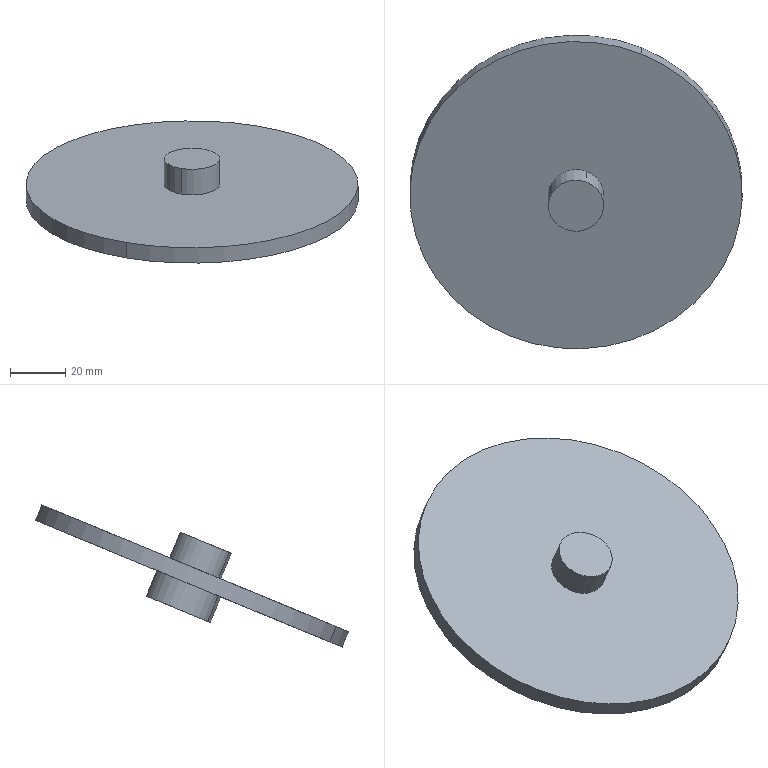Component | SolidWorks | EccentricWheel-2 | 1 solid | 10 faces | box 120 x 113.2 x 51.37 mm | volume 75909 mm3 | cylinder 6 | plane 4 | commonest cylinder face diameters 20 x2 25 x2 120 x2
build123d program:
from build123d import *

# Parameters (mm, degrees)
SKETCH1_R           = 60
BOSS_EXTRUDE1_DEPTH = 6
SKETCH2_R           = 12.5
BOSS_EXTRUDE2_DEPTH = 10
SKETCH3_R           = 10
BOSS_EXTRUDE3_DEPTH = 10


with BuildPart() as part:
    # Sketch1 → Boss-Extrude1 (new body)
    with BuildSketch(Plane.XY):
        Circle(SKETCH1_R)
    extrude(amount=BOSS_EXTRUDE1_DEPTH)

    # Sketch2 → Boss-Extrude2 (add)
    with BuildSketch(Plane(origin=(0, 0, 0), x_dir=(-1, 0, 0), z_dir=(0, 0, -1))):
        Circle(SKETCH2_R)
    extrude(amount=BOSS_EXTRUDE2_DEPTH)

    # Sketch3 → Boss-Extrude3 (add)
    with BuildSketch(Plane.XY.offset(6)):
        Circle(SKETCH3_R)
    extrude(amount=BOSS_EXTRUDE3_DEPTH)


solid = part.part

# Placed as in the assembly
solid = solid.moved(Location((-36.329, 4.513, 6.427), (22.448, 0, 0)))
STEP:
#1=COLOUR_RGB('',0.7922,0.8196,0.9333);
#2=FILL_AREA_STYLE_COLOUR('',#1);
#3=FILL_AREA_STYLE('',(#2));
#4=SURFACE_STYLE_FILL_AREA(#3);
#5=SURFACE_SIDE_STYLE('',(#4));
#6=SURFACE_STYLE_USAGE(.BOTH.,#5);
#7=PRESENTATION_STYLE_ASSIGNMENT((#6));
#8=CARTESIAN_POINT('',(-1.586,-0.3971,0.6971));
#9=VERTEX_POINT('',#8);
#10=CARTESIAN_POINT('',(-1.275,0.2714,0.9733));
#11=VERTEX_POINT('',#10);
#12=CARTESIAN_POINT('',(-1.43,-0.06285,0.8352));
#13=DIRECTION('',(0.,-0.3818,0.9242));
#14=DIRECTION('',(-0.3951,-0.849,-0.3508));
#15=AXIS2_PLACEMENT_3D('',#12,#13,#14);
#16=CIRCLE('',#15,0.3937);
#17=EDGE_CURVE('',#9,#11,#16,.T.);
#18=ORIENTED_EDGE('',*,*,#17,.F.);
#19=CARTESIAN_POINT('',(-1.586,-0.2468,0.3332));
#20=VERTEX_POINT('',#19);
#21=CARTESIAN_POINT('',(-1.586,-0.3971,0.6971));
#22=DIRECTION('',(-0.,0.3818,-0.9242));
#23=VECTOR('',#22,39.37);
#24=LINE('',#21,#23);
#25=EDGE_CURVE('',#9,#20,#24,.T.);
#26=ORIENTED_EDGE('',*,*,#25,.T.);
#27=CARTESIAN_POINT('',(-1.275,0.4218,0.6095));
#28=VERTEX_POINT('',#27);
#29=CARTESIAN_POINT('',(-1.43,0.08749,0.4714));
#30=DIRECTION('',(0.,-0.3818,0.9242));
#31=DIRECTION('',(-0.3951,-0.849,-0.3508));
#32=AXIS2_PLACEMENT_3D('',#29,#30,#31);
#33=CIRCLE('',#32,0.3937);
#34=EDGE_CURVE('',#20,#28,#33,.T.);
#35=ORIENTED_EDGE('',*,*,#34,.T.);
#36=CARTESIAN_POINT('',(-1.275,0.2714,0.9733));
#37=DIRECTION('',(-0.,0.3818,-0.9242));
#38=VECTOR('',#37,39.37);
#39=LINE('',#36,#38);
#40=EDGE_CURVE('',#11,#28,#39,.T.);
#41=ORIENTED_EDGE('',*,*,#40,.F.);
#42=EDGE_LOOP('',(#18,#26,#35,#41));
#43=FACE_OUTER_BOUND('',#42,.T.);
#44=CARTESIAN_POINT('',(-1.43,-0.06285,0.8352));
#45=DIRECTION('',(-0.,0.3818,-0.9242));
#46=DIRECTION('',(0.3951,0.849,0.3508));
#47=AXIS2_PLACEMENT_3D('',#44,#45,#46);
#48=CYLINDRICAL_SURFACE('',#47,0.3937);
#49=ADVANCED_FACE('',(#43),#48,.T.);
#50=CARTESIAN_POINT('',(-1.236,0.7459,0.0618));
#51=VERTEX_POINT('',#50);
#52=CARTESIAN_POINT('',(-1.625,-0.08981,-0.2835));
#53=VERTEX_POINT('',#52);
#54=CARTESIAN_POINT('',(-1.43,0.328,-0.1108));
#55=DIRECTION('',(-0.,0.3818,-0.9242));
#56=DIRECTION('',(0.3951,0.849,0.3508));
#57=AXIS2_PLACEMENT_3D('',#54,#55,#56);
#58=CIRCLE('',#57,0.4921);
#59=EDGE_CURVE('',#51,#53,#58,.T.);
#60=ORIENTED_EDGE('',*,*,#59,.F.);
#61=CARTESIAN_POINT('',(-1.236,0.5955,0.4257));
#62=VERTEX_POINT('',#61);
#63=CARTESIAN_POINT('',(-1.236,0.7459,0.0618));
#64=DIRECTION('',(0.,-0.3818,0.9242));
#65=VECTOR('',#64,39.37);
#66=LINE('',#63,#65);
#67=EDGE_CURVE('',#51,#62,#66,.T.);
#68=ORIENTED_EDGE('',*,*,#67,.T.);
#69=CARTESIAN_POINT('',(-1.625,-0.2401,0.0804));
#70=VERTEX_POINT('',#69);
#71=CARTESIAN_POINT('',(-1.43,0.1777,0.253));
#72=DIRECTION('',(-0.,0.3818,-0.9242));
#73=DIRECTION('',(0.3951,0.849,0.3508));
#74=AXIS2_PLACEMENT_3D('',#71,#72,#73);
#75=CIRCLE('',#74,0.4921);
#76=EDGE_CURVE('',#62,#70,#75,.T.);
#77=ORIENTED_EDGE('',*,*,#76,.T.);
#78=CARTESIAN_POINT('',(-1.625,-0.08981,-0.2835));
#79=DIRECTION('',(0.,-0.3818,0.9242));
#80=VECTOR('',#79,39.37);
#81=LINE('',#78,#80);
#82=EDGE_CURVE('',#53,#70,#81,.T.);
#83=ORIENTED_EDGE('',*,*,#82,.F.);
#84=EDGE_LOOP('',(#60,#68,#77,#83));
#85=FACE_OUTER_BOUND('',#84,.T.);
#86=CARTESIAN_POINT('',(-1.43,0.328,-0.1108));
#87=DIRECTION('',(0.,-0.3818,0.9242));
#88=DIRECTION('',(-0.3951,-0.849,-0.3508));
#89=AXIS2_PLACEMENT_3D('',#86,#87,#88);
#90=CYLINDRICAL_SURFACE('',#89,0.4921);
#91=ADVANCED_FACE('',(#85),#90,.T.);
#92=CARTESIAN_POINT('',(-2.364,-1.918,-0.3573));
#93=VERTEX_POINT('',#92);
#94=CARTESIAN_POINT('',(-0.497,2.093,1.3));
#95=VERTEX_POINT('',#94);
#96=CARTESIAN_POINT('',(-1.43,0.08749,0.4714));
#97=DIRECTION('',(0.,-0.3818,0.9242));
#98=DIRECTION('',(-0.3951,-0.849,-0.3508));
#99=AXIS2_PLACEMENT_3D('',#96,#97,#98);
#100=CIRCLE('',#99,2.362);
#101=EDGE_CURVE('',#93,#95,#100,.T.);
#102=ORIENTED_EDGE('',*,*,#101,.F.);
#103=CARTESIAN_POINT('',(-2.364,-1.828,-0.5756));
#104=VERTEX_POINT('',#103);
#105=CARTESIAN_POINT('',(-2.364,-1.918,-0.3573));
#106=DIRECTION('',(-0.,0.3818,-0.9242));
#107=VECTOR('',#106,39.37);
#108=LINE('',#105,#107);
#109=EDGE_CURVE('',#93,#104,#108,.T.);
#110=ORIENTED_EDGE('',*,*,#109,.T.);
#111=CARTESIAN_POINT('',(-0.497,2.183,1.082));
#112=VERTEX_POINT('',#111);
#113=CARTESIAN_POINT('',(-1.43,0.1777,0.253));
#114=DIRECTION('',(0.,-0.3818,0.9242));
#115=DIRECTION('',(-0.3951,-0.849,-0.3508));
#116=AXIS2_PLACEMENT_3D('',#113,#114,#115);
#117=CIRCLE('',#116,2.362);
#118=EDGE_CURVE('',#104,#112,#117,.T.);
#119=ORIENTED_EDGE('',*,*,#118,.T.);
#120=CARTESIAN_POINT('',(-0.497,2.093,1.3));
#121=DIRECTION('',(-0.,0.3818,-0.9242));
#122=VECTOR('',#121,39.37);
#123=LINE('',#120,#122);
#124=EDGE_CURVE('',#95,#112,#123,.T.);
#125=ORIENTED_EDGE('',*,*,#124,.F.);
#126=EDGE_LOOP('',(#102,#110,#119,#125));
#127=FACE_OUTER_BOUND('',#126,.T.);
#128=CARTESIAN_POINT('',(-1.43,0.08749,0.4714));
#129=DIRECTION('',(-0.,0.3818,-0.9242));
#130=DIRECTION('',(0.3951,0.849,0.3508));
#131=AXIS2_PLACEMENT_3D('',#128,#129,#130);
#132=CYLINDRICAL_SURFACE('',#131,2.362);
#133=ADVANCED_FACE('',(#127),#132,.T.);
#134=ORIENTED_EDGE('',*,*,#109,.F.);
#135=CARTESIAN_POINT('',(-1.43,0.08749,0.4714));
#136=DIRECTION('',(0.,-0.3818,0.9242));
#137=DIRECTION('',(-0.3951,-0.849,-0.3508));
#138=AXIS2_PLACEMENT_3D('',#135,#136,#137);
#139=CIRCLE('',#138,2.362);
#140=EDGE_CURVE('',#95,#93,#139,.T.);
#141=ORIENTED_EDGE('',*,*,#140,.F.);
#142=ORIENTED_EDGE('',*,*,#124,.T.);
#143=CARTESIAN_POINT('',(-1.43,0.1777,0.253));
#144=DIRECTION('',(0.,-0.3818,0.9242));
#145=DIRECTION('',(-0.3951,-0.849,-0.3508));
#146=AXIS2_PLACEMENT_3D('',#143,#144,#145);
#147=CIRCLE('',#146,2.362);
#148=EDGE_CURVE('',#112,#104,#147,.T.);
#149=ORIENTED_EDGE('',*,*,#148,.T.);
#150=EDGE_LOOP('',(#134,#141,#142,#149));
#151=FACE_OUTER_BOUND('',#150,.T.);
#152=CARTESIAN_POINT('',(-1.43,0.08749,0.4714));
#153=DIRECTION('',(-0.,0.3818,-0.9242));
#154=DIRECTION('',(0.3951,0.849,0.3508));
#155=AXIS2_PLACEMENT_3D('',#152,#153,#154);
#156=CYLINDRICAL_SURFACE('',#155,2.362);
#157=ADVANCED_FACE('',(#151),#156,.T.);
#158=CARTESIAN_POINT('',(-1.43,0.08749,0.4714));
#159=DIRECTION('',(0.,-0.3818,0.9242));
#160=DIRECTION('',(-0.3951,-0.849,-0.3508));
#161=AXIS2_PLACEMENT_3D('',#158,#159,#160);
#162=CIRCLE('',#161,0.3937);
#163=EDGE_CURVE('',#28,#20,#162,.T.);
#164=ORIENTED_EDGE('',*,*,#163,.F.);
#165=ORIENTED_EDGE('',*,*,#34,.F.);
#166=EDGE_LOOP('',(#164,#165));
#167=FACE_BOUND('',#166,.T.);
#168=ORIENTED_EDGE('',*,*,#140,.T.);
#169=ORIENTED_EDGE('',*,*,#101,.T.);
#170=EDGE_LOOP('',(#168,#169));
#171=FACE_OUTER_BOUND('',#170,.T.);
#172=CARTESIAN_POINT('',(-1.43,0.08749,0.4714));
#173=DIRECTION('',(0.,-0.3818,0.9242));
#174=DIRECTION('',(-0.3951,-0.849,-0.3508));
#175=AXIS2_PLACEMENT_3D('',#172,#173,#174);
#176=PLANE('',#175);
#177=ADVANCED_FACE('',(#167,#171),#176,.T.);
#178=CARTESIAN_POINT('',(-1.43,0.1777,0.253));
#179=DIRECTION('',(-0.,0.3818,-0.9242));
#180=DIRECTION('',(0.3951,0.849,0.3508));
#181=AXIS2_PLACEMENT_3D('',#178,#179,#180);
#182=CIRCLE('',#181,0.4921);
#183=EDGE_CURVE('',#70,#62,#182,.T.);
#184=ORIENTED_EDGE('',*,*,#183,.F.);
#185=ORIENTED_EDGE('',*,*,#76,.F.);
#186=EDGE_LOOP('',(#184,#185));
#187=FACE_BOUND('',#186,.T.);
#188=ORIENTED_EDGE('',*,*,#148,.F.);
#189=ORIENTED_EDGE('',*,*,#118,.F.);
#190=EDGE_LOOP('',(#188,#189));
#191=FACE_OUTER_BOUND('',#190,.T.);
#192=CARTESIAN_POINT('',(-1.43,0.1777,0.253));
#193=DIRECTION('',(0.,-0.3818,0.9242));
#194=DIRECTION('',(-0.3951,-0.849,-0.3508));
#195=AXIS2_PLACEMENT_3D('',#192,#193,#194);
#196=PLANE('',#195);
#197=ADVANCED_FACE('',(#187,#191),#196,.F.);
#198=ORIENTED_EDGE('',*,*,#67,.F.);
#199=CARTESIAN_POINT('',(-1.43,0.328,-0.1108));
#200=DIRECTION('',(-0.,0.3818,-0.9242));
#201=DIRECTION('',(0.3951,0.849,0.3508));
#202=AXIS2_PLACEMENT_3D('',#199,#200,#201);
#203=CIRCLE('',#202,0.4921);
#204=EDGE_CURVE('',#53,#51,#203,.T.);
#205=ORIENTED_EDGE('',*,*,#204,.F.);
#206=ORIENTED_EDGE('',*,*,#82,.T.);
#207=ORIENTED_EDGE('',*,*,#183,.T.);
#208=EDGE_LOOP('',(#198,#205,#206,#207));
#209=FACE_OUTER_BOUND('',#208,.T.);
#210=CARTESIAN_POINT('',(-1.43,0.328,-0.1108));
#211=DIRECTION('',(0.,-0.3818,0.9242));
#212=DIRECTION('',(-0.3951,-0.849,-0.3508));
#213=AXIS2_PLACEMENT_3D('',#210,#211,#212);
#214=CYLINDRICAL_SURFACE('',#213,0.4921);
#215=ADVANCED_FACE('',(#209),#214,.T.);
#216=ORIENTED_EDGE('',*,*,#204,.T.);
#217=ORIENTED_EDGE('',*,*,#59,.T.);
#218=EDGE_LOOP('',(#216,#217));
#219=FACE_OUTER_BOUND('',#218,.T.);
#220=CARTESIAN_POINT('',(-1.43,0.328,-0.1108));
#221=DIRECTION('',(-0.,0.3818,-0.9242));
#222=DIRECTION('',(0.3951,0.849,0.3508));
#223=AXIS2_PLACEMENT_3D('',#220,#221,#222);
#224=PLANE('',#223);
#225=ADVANCED_FACE('',(#219),#224,.T.);
#226=ORIENTED_EDGE('',*,*,#25,.F.);
#227=CARTESIAN_POINT('',(-1.43,-0.06285,0.8352));
#228=DIRECTION('',(0.,-0.3818,0.9242));
#229=DIRECTION('',(-0.3951,-0.849,-0.3508));
#230=AXIS2_PLACEMENT_3D('',#227,#228,#229);
#231=CIRCLE('',#230,0.3937);
#232=EDGE_CURVE('',#11,#9,#231,.T.);
#233=ORIENTED_EDGE('',*,*,#232,.F.);
#234=ORIENTED_EDGE('',*,*,#40,.T.);
#235=ORIENTED_EDGE('',*,*,#163,.T.);
#236=EDGE_LOOP('',(#226,#233,#234,#235));
#237=FACE_OUTER_BOUND('',#236,.T.);
#238=CARTESIAN_POINT('',(-1.43,-0.06285,0.8352));
#239=DIRECTION('',(-0.,0.3818,-0.9242));
#240=DIRECTION('',(0.3951,0.849,0.3508));
#241=AXIS2_PLACEMENT_3D('',#238,#239,#240);
#242=CYLINDRICAL_SURFACE('',#241,0.3937);
#243=ADVANCED_FACE('',(#237),#242,.T.);
#244=ORIENTED_EDGE('',*,*,#232,.T.);
#245=ORIENTED_EDGE('',*,*,#17,.T.);
#246=EDGE_LOOP('',(#244,#245));
#247=FACE_OUTER_BOUND('',#246,.T.);
#248=CARTESIAN_POINT('',(-1.43,-0.06285,0.8352));
#249=DIRECTION('',(0.,-0.3818,0.9242));
#250=DIRECTION('',(-0.3951,-0.849,-0.3508));
#251=AXIS2_PLACEMENT_3D('',#248,#249,#250);
#252=PLANE('',#251);
#253=ADVANCED_FACE('',(#247),#252,.T.);
#254=CLOSED_SHELL('',(#49,#91,#133,#157,#177,#197,#215,#225,#243,#253));
#255=MANIFOLD_SOLID_BREP('',#254);
#256=STYLED_ITEM('',(#7),#255);
#257=PRESENTATION_LAYER_ASSIGNMENT('','',(#256));
#258=CARTESIAN_POINT('',(0.,0.,0.));
#259=DIRECTION('',(0.,0.,1.));
#260=DIRECTION('',(1.,0.,0.));
#261=AXIS2_PLACEMENT_3D('',#258,#259,#260);
#262=(LENGTH_UNIT()NAMED_UNIT(*)SI_UNIT($,.METRE.));
#263=LENGTH_MEASURE_WITH_UNIT(LENGTH_MEASURE(0.0254),#262);
#264=DIMENSIONAL_EXPONENTS(1.,0.,0.,0.,0.,0.,0.);
#265=(CONVERSION_BASED_UNIT('',#263)LENGTH_UNIT()NAMED_UNIT(#264));
#266=UNCERTAINTY_MEASURE_WITH_UNIT(LENGTH_MEASURE(0.00001),#265,'','');
#267=(NAMED_UNIT(*)PLANE_ANGLE_UNIT()SI_UNIT($,.RADIAN.));
#268=(NAMED_UNIT(*)SI_UNIT($,.STERADIAN.)SOLID_ANGLE_UNIT());
#269=(GEOMETRIC_REPRESENTATION_CONTEXT(3)GLOBAL_UNCERTAINTY_ASSIGNED_CONTEXT((#266))GLOBAL_UNIT_ASSIGNED_CONTEXT((#265,#267,#268))REPRESENTATION_CONTEXT('',''));
#270=ADVANCED_BREP_SHAPE_REPRESENTATION('',(#255,#261),#269);
#271=(LENGTH_UNIT()NAMED_UNIT(*)SI_UNIT($,.METRE.));
#272=LENGTH_MEASURE_WITH_UNIT(LENGTH_MEASURE(0.0254),#271);
#273=DIMENSIONAL_EXPONENTS(1.,0.,0.,0.,0.,0.,0.);
#274=(CONVERSION_BASED_UNIT('',#272)LENGTH_UNIT()NAMED_UNIT(#273));
#275=UNCERTAINTY_MEASURE_WITH_UNIT(LENGTH_MEASURE(0.00001),#274,'','');
#276=(NAMED_UNIT(*)PLANE_ANGLE_UNIT()SI_UNIT($,.RADIAN.));
#277=(NAMED_UNIT(*)SI_UNIT($,.STERADIAN.)SOLID_ANGLE_UNIT());
#278=(GEOMETRIC_REPRESENTATION_CONTEXT(3)GLOBAL_UNCERTAINTY_ASSIGNED_CONTEXT((#275))GLOBAL_UNIT_ASSIGNED_CONTEXT((#274,#276,#277))REPRESENTATION_CONTEXT('',''));
#279=MECHANICAL_DESIGN_GEOMETRIC_PRESENTATION_REPRESENTATION('',(#256),#278);